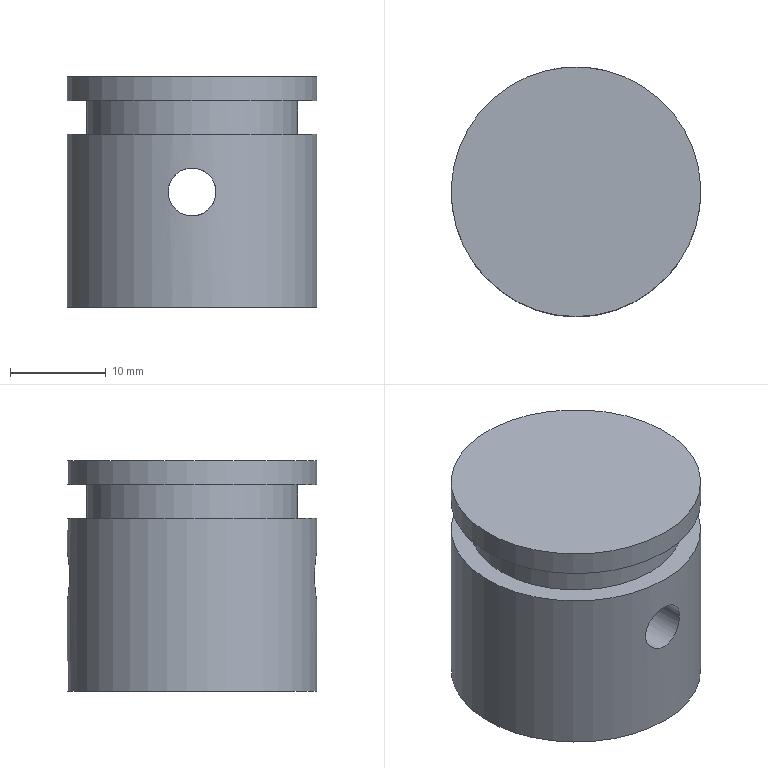Component | NX | PISTON | 1 solid | 12 faces | volume 7592 mm3 | cylinder 6 | plane 5 | torus 1 | commonest cylinder face diameters 26 x2 5 x2 17 x1 22 x1